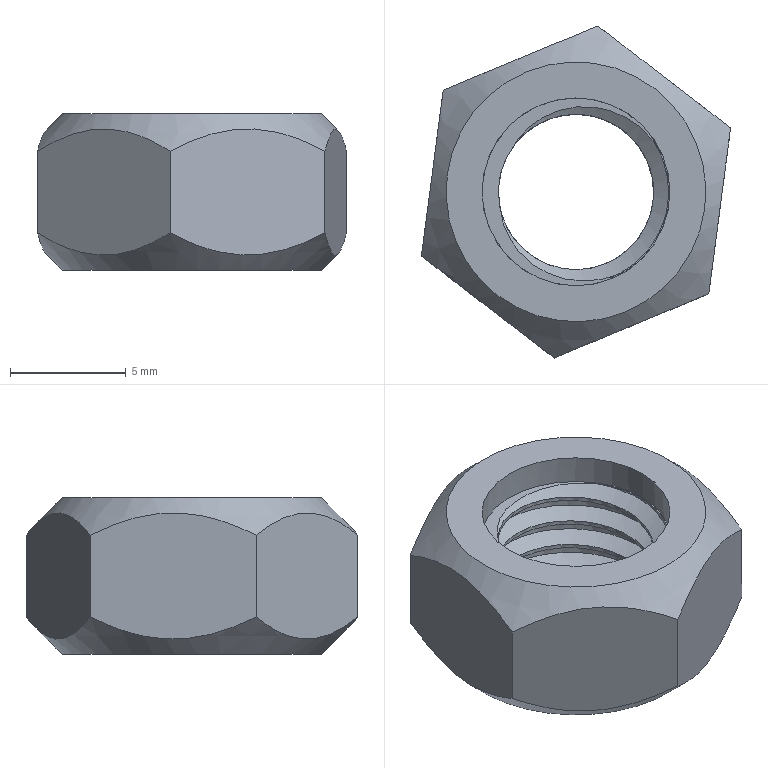Component | NX | NUT | 1 solid | 16 faces | volume 569 mm3 | plane 9 | cylinder 3 | cone 2 | spline 2 | commonest cylinder face diameters 6.7 x1 8 x1 8.1 x1